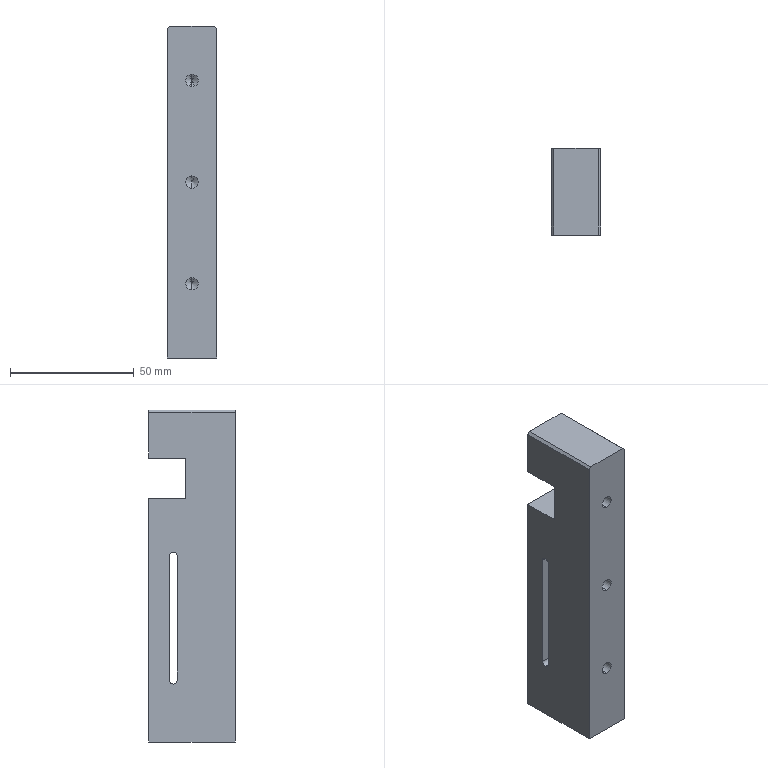Component | SolidWorks | J-TRD899MINI-2213-01DesiccantPressingSupportPlate-4 | 1 solid | 48 faces | box 20 x 35 x 134 mm | volume 81968 mm3 | cylinder 18 | cone 16 | plane 14 | commonest cylinder face diameters 5 x10 3.2 x4 6.8 x4 | material 6061
build123d program:
from build123d import *

# Parameters (mm, degrees)
SKETCH1_W             = 134
SKETCH1_H             = 35
BOSS_EXTRUDE1_DEPTH   = 20
M8_TAPPED_HOLE1_D     = 6.8
M8_TAPPED_HOLE1_DEPTH = 23.75
M8_TAPPED_HOLE1_TIP   = 2.043
CUT_EXTRUDE1_DEPTH    = 73.078
M6_TAPPED_HOLE3_D     = 5
M6_TAPPED_HOLE3_DEPTH = 18
M6_TAPPED_HOLE3_TIP   = 1.502
M6_TAPPED_HOLE4_D     = 5
M6_TAPPED_HOLE4_DEPTH = 18
M6_TAPPED_HOLE4_TIP   = 1.502
SKETCH13_W            = 16.2
SKETCH13_H            = 15
CUT_EXTRUDE2_DEPTH    = 73.078
CHAMFER1_SIZE         = 1


with BuildPart() as part:
    # Sketch1 → Boss-Extrude1 (new body)
    with BuildSketch(Plane(origin=(0, 0, 0), x_dir=(0, 0, -1), z_dir=(1, 0, 0))):
        Rectangle(SKETCH1_W, SKETCH1_H)
    extrude(amount=BOSS_EXTRUDE1_DEPTH)

    # M8 Tapped Hole1
    with Locations(Plane(origin=(0, 0, -67), x_dir=(-1, 0, 0), z_dir=(0, 0, -1))):
        with Locations((-10, 9), (-10, -9)):
            Hole(M8_TAPPED_HOLE1_D / 2, depth=M8_TAPPED_HOLE1_DEPTH)
            with Locations((0, 0, -(M8_TAPPED_HOLE1_DEPTH + M8_TAPPED_HOLE1_TIP / 2))):  # 118° drill point
                Cone(0, M8_TAPPED_HOLE1_D / 2, M8_TAPPED_HOLE1_TIP, mode=Mode.SUBTRACT)

    # Sketch4 → Cut-Extrude1 (cut, through all)
    with BuildSketch(Plane(origin=(20, 0, 0), x_dir=(0, 0, -1), z_dir=(1, 0, 0))):
        with BuildLine():
            Line((-8, 9.1), (42, 9.1))
            ThreePointArc((42, 9.1), (43.6, 7.5), (42, 5.9))
            Line((42, 5.9), (-8, 5.9))
            ThreePointArc((-8, 5.9), (-9.6, 7.5), (-8, 9.1))
        make_face()
    extrude(amount=-CUT_EXTRUDE1_DEPTH, mode=Mode.SUBTRACT)

    # M6 Tapped Hole3
    with Locations(Plane(origin=(0, -17.5, 0), x_dir=(-1, 0, 0), z_dir=(0, -1, 0))):
        with Locations((-10, 37), (-10, -4), (-10, -45)):
            Hole(M6_TAPPED_HOLE3_D / 2, depth=M6_TAPPED_HOLE3_DEPTH)
            with Locations((0, 0, -(M6_TAPPED_HOLE3_DEPTH + M6_TAPPED_HOLE3_TIP / 2))):  # 118° drill point
                Cone(0, M6_TAPPED_HOLE3_D / 2, M6_TAPPED_HOLE3_TIP, mode=Mode.SUBTRACT)

    # M6 Tapped Hole4
    with Locations(Plane(origin=(0, 17.5, 0), x_dir=(1, 0, 0), z_dir=(0, 1, 0))):
        with Locations((10, -61), (10, -18)):
            Hole(M6_TAPPED_HOLE4_D / 2, depth=M6_TAPPED_HOLE4_DEPTH)
            with Locations((0, 0, -(M6_TAPPED_HOLE4_DEPTH + M6_TAPPED_HOLE4_TIP / 2))):  # 118° drill point
                Cone(0, M6_TAPPED_HOLE4_D / 2, M6_TAPPED_HOLE4_TIP, mode=Mode.SUBTRACT)

    # Sketch13 → Cut-Extrude2 (cut, through all)
    with BuildSketch(Plane(origin=(20, 0, 0), x_dir=(0, 0, -1), z_dir=(1, 0, 0))):
        with Locations((-39.5, 10)):
            Rectangle(SKETCH13_W, SKETCH13_H)
    extrude(amount=-CUT_EXTRUDE2_DEPTH, mode=Mode.SUBTRACT)

    # Chamfer1
    chamfer1_edges = [part.edges().sort_by_distance(p)[0] for p in [
        (20, 0, 67),
        (0, 0, 67),
    ]]
    chamfer(chamfer1_edges, length=CHAMFER1_SIZE)


solid = part.part

# Placed as in the assembly
solid = solid.moved(Location((-131.663, 8.496, 152), (0, 0, 0)))